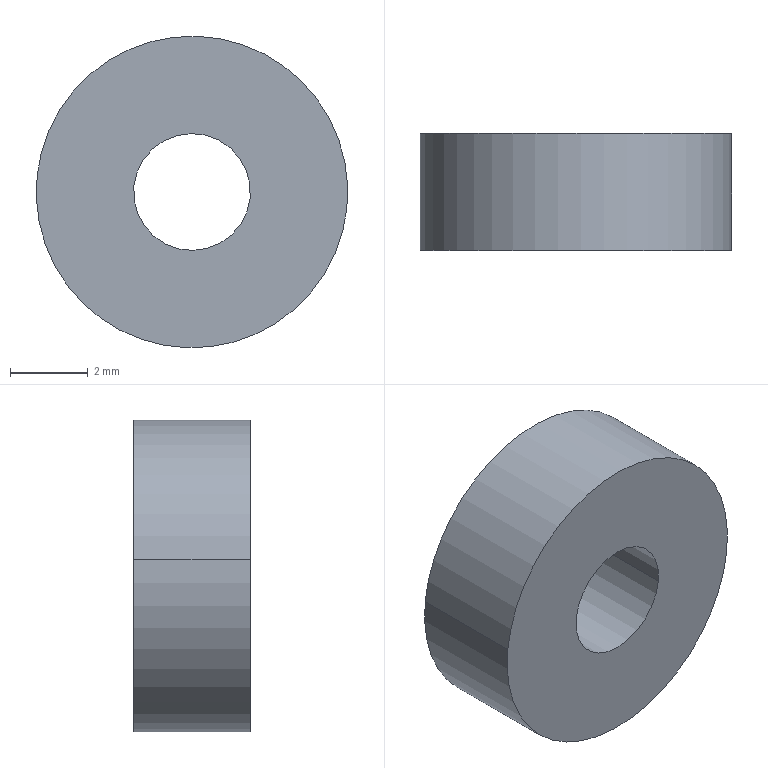Component | SolidWorks | Roller-12 | 1 solid | 6 faces | box 8 x 3 x 8 mm | volume 130 mm3 | cylinder 4 | plane 2 | commonest cylinder face diameters 3 x2 8 x2
build123d program:
from build123d import *

# Parameters (mm, degrees)
SKETCH1_R           = 4
SKETCH1_R_2         = 1.5
BOSS_EXTRUDE1_DEPTH = 3


with BuildPart() as part:
    # Sketch1 → Boss-Extrude1 (new body)
    with BuildSketch(Plane.XY):
        Circle(SKETCH1_R)
        Circle(SKETCH1_R_2, mode=Mode.SUBTRACT)
    extrude(amount=BOSS_EXTRUDE1_DEPTH)


solid = part.part

# Placed as in the assembly
solid = solid.moved(Location((-16.097, 11.517, 56), (90, 0, 0)))
STEP:
#1=COLOUR_RGB('',0.7922,0.8196,0.9333);
#2=FILL_AREA_STYLE_COLOUR('',#1);
#3=FILL_AREA_STYLE('',(#2));
#4=SURFACE_STYLE_FILL_AREA(#3);
#5=SURFACE_SIDE_STYLE('',(#4));
#6=SURFACE_STYLE_USAGE(.BOTH.,#5);
#7=PRESENTATION_STYLE_ASSIGNMENT((#6));
#8=CARTESIAN_POINT('',(-0.6924,0.3353,2.211));
#9=VERTEX_POINT('',#8);
#10=CARTESIAN_POINT('',(-0.575,0.3353,2.198));
#11=VERTEX_POINT('',#10);
#12=CARTESIAN_POINT('',(-0.6337,0.3353,2.205));
#13=DIRECTION('',(0.,-1.,0.));
#14=DIRECTION('',(0.9943,0.,-0.107));
#15=AXIS2_PLACEMENT_3D('',#12,#13,#14);
#16=CIRCLE('',#15,0.05906);
#17=EDGE_CURVE('',#9,#11,#16,.T.);
#18=ORIENTED_EDGE('',*,*,#17,.T.);
#19=CARTESIAN_POINT('',(-0.575,0.4534,2.198));
#20=VERTEX_POINT('',#19);
#21=CARTESIAN_POINT('',(-0.575,0.3353,2.198));
#22=DIRECTION('',(0.,1.,0.));
#23=VECTOR('',#22,39.37);
#24=LINE('',#21,#23);
#25=EDGE_CURVE('',#11,#20,#24,.T.);
#26=ORIENTED_EDGE('',*,*,#25,.T.);
#27=CARTESIAN_POINT('',(-0.6924,0.4534,2.211));
#28=VERTEX_POINT('',#27);
#29=CARTESIAN_POINT('',(-0.6337,0.4534,2.205));
#30=DIRECTION('',(0.,-1.,0.));
#31=DIRECTION('',(0.9943,0.,-0.107));
#32=AXIS2_PLACEMENT_3D('',#29,#30,#31);
#33=CIRCLE('',#32,0.05906);
#34=EDGE_CURVE('',#28,#20,#33,.T.);
#35=ORIENTED_EDGE('',*,*,#34,.F.);
#36=CARTESIAN_POINT('',(-0.6924,0.3353,2.211));
#37=DIRECTION('',(0.,1.,0.));
#38=VECTOR('',#37,39.37);
#39=LINE('',#36,#38);
#40=EDGE_CURVE('',#9,#28,#39,.T.);
#41=ORIENTED_EDGE('',*,*,#40,.F.);
#42=EDGE_LOOP('',(#18,#26,#35,#41));
#43=FACE_OUTER_BOUND('',#42,.T.);
#44=CARTESIAN_POINT('',(-0.6337,0.3353,2.205));
#45=DIRECTION('',(0.,1.,0.));
#46=DIRECTION('',(-0.9943,0.,0.107));
#47=AXIS2_PLACEMENT_3D('',#44,#45,#46);
#48=CYLINDRICAL_SURFACE('',#47,0.05906);
#49=ADVANCED_FACE('',(#43),#48,.F.);
#50=CARTESIAN_POINT('',(-0.4772,0.3353,2.188));
#51=VERTEX_POINT('',#50);
#52=CARTESIAN_POINT('',(-0.7903,0.3353,2.222));
#53=VERTEX_POINT('',#52);
#54=CARTESIAN_POINT('',(-0.6337,0.3353,2.205));
#55=DIRECTION('',(0.,-1.,0.));
#56=DIRECTION('',(0.9943,0.,-0.107));
#57=AXIS2_PLACEMENT_3D('',#54,#55,#56);
#58=CIRCLE('',#57,0.1575);
#59=EDGE_CURVE('',#51,#53,#58,.T.);
#60=ORIENTED_EDGE('',*,*,#59,.F.);
#61=CARTESIAN_POINT('',(-0.4772,0.4534,2.188));
#62=VERTEX_POINT('',#61);
#63=CARTESIAN_POINT('',(-0.4772,0.3353,2.188));
#64=DIRECTION('',(0.,1.,0.));
#65=VECTOR('',#64,39.37);
#66=LINE('',#63,#65);
#67=EDGE_CURVE('',#51,#62,#66,.T.);
#68=ORIENTED_EDGE('',*,*,#67,.T.);
#69=CARTESIAN_POINT('',(-0.7903,0.4534,2.222));
#70=VERTEX_POINT('',#69);
#71=CARTESIAN_POINT('',(-0.6337,0.4534,2.205));
#72=DIRECTION('',(0.,-1.,0.));
#73=DIRECTION('',(0.9943,0.,-0.107));
#74=AXIS2_PLACEMENT_3D('',#71,#72,#73);
#75=CIRCLE('',#74,0.1575);
#76=EDGE_CURVE('',#62,#70,#75,.T.);
#77=ORIENTED_EDGE('',*,*,#76,.T.);
#78=CARTESIAN_POINT('',(-0.7903,0.3353,2.222));
#79=DIRECTION('',(0.,1.,0.));
#80=VECTOR('',#79,39.37);
#81=LINE('',#78,#80);
#82=EDGE_CURVE('',#53,#70,#81,.T.);
#83=ORIENTED_EDGE('',*,*,#82,.F.);
#84=EDGE_LOOP('',(#60,#68,#77,#83));
#85=FACE_OUTER_BOUND('',#84,.T.);
#86=CARTESIAN_POINT('',(-0.6337,0.3353,2.205));
#87=DIRECTION('',(0.,1.,0.));
#88=DIRECTION('',(-0.9943,0.,0.107));
#89=AXIS2_PLACEMENT_3D('',#86,#87,#88);
#90=CYLINDRICAL_SURFACE('',#89,0.1575);
#91=ADVANCED_FACE('',(#85),#90,.T.);
#92=CARTESIAN_POINT('',(-0.6337,0.3353,2.205));
#93=DIRECTION('',(0.,-1.,0.));
#94=DIRECTION('',(0.9943,0.,-0.107));
#95=AXIS2_PLACEMENT_3D('',#92,#93,#94);
#96=CIRCLE('',#95,0.1575);
#97=EDGE_CURVE('',#53,#51,#96,.T.);
#98=ORIENTED_EDGE('',*,*,#97,.T.);
#99=ORIENTED_EDGE('',*,*,#59,.T.);
#100=EDGE_LOOP('',(#98,#99));
#101=FACE_OUTER_BOUND('',#100,.T.);
#102=ORIENTED_EDGE('',*,*,#17,.F.);
#103=CARTESIAN_POINT('',(-0.6337,0.3353,2.205));
#104=DIRECTION('',(0.,-1.,0.));
#105=DIRECTION('',(0.9943,0.,-0.107));
#106=AXIS2_PLACEMENT_3D('',#103,#104,#105);
#107=CIRCLE('',#106,0.05906);
#108=EDGE_CURVE('',#11,#9,#107,.T.);
#109=ORIENTED_EDGE('',*,*,#108,.F.);
#110=EDGE_LOOP('',(#102,#109));
#111=FACE_BOUND('',#110,.T.);
#112=CARTESIAN_POINT('',(-0.6337,0.3353,2.205));
#113=DIRECTION('',(0.,-1.,0.));
#114=DIRECTION('',(0.9943,0.,-0.107));
#115=AXIS2_PLACEMENT_3D('',#112,#113,#114);
#116=PLANE('',#115);
#117=ADVANCED_FACE('',(#101,#111),#116,.T.);
#118=CARTESIAN_POINT('',(-0.6337,0.4534,2.205));
#119=DIRECTION('',(0.,-1.,0.));
#120=DIRECTION('',(0.9943,0.,-0.107));
#121=AXIS2_PLACEMENT_3D('',#118,#119,#120);
#122=CIRCLE('',#121,0.1575);
#123=EDGE_CURVE('',#70,#62,#122,.T.);
#124=ORIENTED_EDGE('',*,*,#123,.F.);
#125=ORIENTED_EDGE('',*,*,#76,.F.);
#126=EDGE_LOOP('',(#124,#125));
#127=FACE_OUTER_BOUND('',#126,.T.);
#128=ORIENTED_EDGE('',*,*,#34,.T.);
#129=CARTESIAN_POINT('',(-0.6337,0.4534,2.205));
#130=DIRECTION('',(0.,-1.,0.));
#131=DIRECTION('',(0.9943,0.,-0.107));
#132=AXIS2_PLACEMENT_3D('',#129,#130,#131);
#133=CIRCLE('',#132,0.05906);
#134=EDGE_CURVE('',#20,#28,#133,.T.);
#135=ORIENTED_EDGE('',*,*,#134,.T.);
#136=EDGE_LOOP('',(#128,#135));
#137=FACE_BOUND('',#136,.T.);
#138=CARTESIAN_POINT('',(-0.6337,0.4534,2.205));
#139=DIRECTION('',(0.,-1.,0.));
#140=DIRECTION('',(0.9943,0.,-0.107));
#141=AXIS2_PLACEMENT_3D('',#138,#139,#140);
#142=PLANE('',#141);
#143=ADVANCED_FACE('',(#127,#137),#142,.F.);
#144=ORIENTED_EDGE('',*,*,#67,.F.);
#145=ORIENTED_EDGE('',*,*,#97,.F.);
#146=ORIENTED_EDGE('',*,*,#82,.T.);
#147=ORIENTED_EDGE('',*,*,#123,.T.);
#148=EDGE_LOOP('',(#144,#145,#146,#147));
#149=FACE_OUTER_BOUND('',#148,.T.);
#150=CARTESIAN_POINT('',(-0.6337,0.3353,2.205));
#151=DIRECTION('',(0.,1.,0.));
#152=DIRECTION('',(-0.9943,0.,0.107));
#153=AXIS2_PLACEMENT_3D('',#150,#151,#152);
#154=CYLINDRICAL_SURFACE('',#153,0.1575);
#155=ADVANCED_FACE('',(#149),#154,.T.);
#156=ORIENTED_EDGE('',*,*,#25,.F.);
#157=ORIENTED_EDGE('',*,*,#108,.T.);
#158=ORIENTED_EDGE('',*,*,#40,.T.);
#159=ORIENTED_EDGE('',*,*,#134,.F.);
#160=EDGE_LOOP('',(#156,#157,#158,#159));
#161=FACE_OUTER_BOUND('',#160,.T.);
#162=CARTESIAN_POINT('',(-0.6337,0.3353,2.205));
#163=DIRECTION('',(0.,1.,0.));
#164=DIRECTION('',(-0.9943,0.,0.107));
#165=AXIS2_PLACEMENT_3D('',#162,#163,#164);
#166=CYLINDRICAL_SURFACE('',#165,0.05906);
#167=ADVANCED_FACE('',(#161),#166,.F.);
#168=CLOSED_SHELL('',(#49,#91,#117,#143,#155,#167));
#169=MANIFOLD_SOLID_BREP('',#168);
#170=STYLED_ITEM('',(#7),#169);
#171=(LENGTH_UNIT()NAMED_UNIT(*)SI_UNIT($,.METRE.));
#172=LENGTH_MEASURE_WITH_UNIT(LENGTH_MEASURE(0.0254),#171);
#173=DIMENSIONAL_EXPONENTS(1.,0.,0.,0.,0.,0.,0.);
#174=(CONVERSION_BASED_UNIT('',#172)LENGTH_UNIT()NAMED_UNIT(#173));
#175=UNCERTAINTY_MEASURE_WITH_UNIT(LENGTH_MEASURE(0.00001),#174,'','');
#176=(NAMED_UNIT(*)PLANE_ANGLE_UNIT()SI_UNIT($,.RADIAN.));
#177=(NAMED_UNIT(*)SI_UNIT($,.STERADIAN.)SOLID_ANGLE_UNIT());
#178=(GEOMETRIC_REPRESENTATION_CONTEXT(3)GLOBAL_UNCERTAINTY_ASSIGNED_CONTEXT((#175))GLOBAL_UNIT_ASSIGNED_CONTEXT((#174,#176,#177))REPRESENTATION_CONTEXT('',''));
#179=MECHANICAL_DESIGN_GEOMETRIC_PRESENTATION_REPRESENTATION('',(#170),#178);
#180=PRESENTATION_LAYER_ASSIGNMENT('','',(#170));
#181=CARTESIAN_POINT('',(0.,0.,0.));
#182=DIRECTION('',(0.,0.,1.));
#183=DIRECTION('',(1.,0.,0.));
#184=AXIS2_PLACEMENT_3D('',#181,#182,#183);
#185=(LENGTH_UNIT()NAMED_UNIT(*)SI_UNIT($,.METRE.));
#186=LENGTH_MEASURE_WITH_UNIT(LENGTH_MEASURE(0.0254),#185);
#187=DIMENSIONAL_EXPONENTS(1.,0.,0.,0.,0.,0.,0.);
#188=(CONVERSION_BASED_UNIT('',#186)LENGTH_UNIT()NAMED_UNIT(#187));
#189=UNCERTAINTY_MEASURE_WITH_UNIT(LENGTH_MEASURE(0.00001),#188,'','');
#190=(NAMED_UNIT(*)PLANE_ANGLE_UNIT()SI_UNIT($,.RADIAN.));
#191=(NAMED_UNIT(*)SI_UNIT($,.STERADIAN.)SOLID_ANGLE_UNIT());
#192=(GEOMETRIC_REPRESENTATION_CONTEXT(3)GLOBAL_UNCERTAINTY_ASSIGNED_CONTEXT((#189))GLOBAL_UNIT_ASSIGNED_CONTEXT((#188,#190,#191))REPRESENTATION_CONTEXT('',''));
#193=ADVANCED_BREP_SHAPE_REPRESENTATION('',(#169,#184),#192);